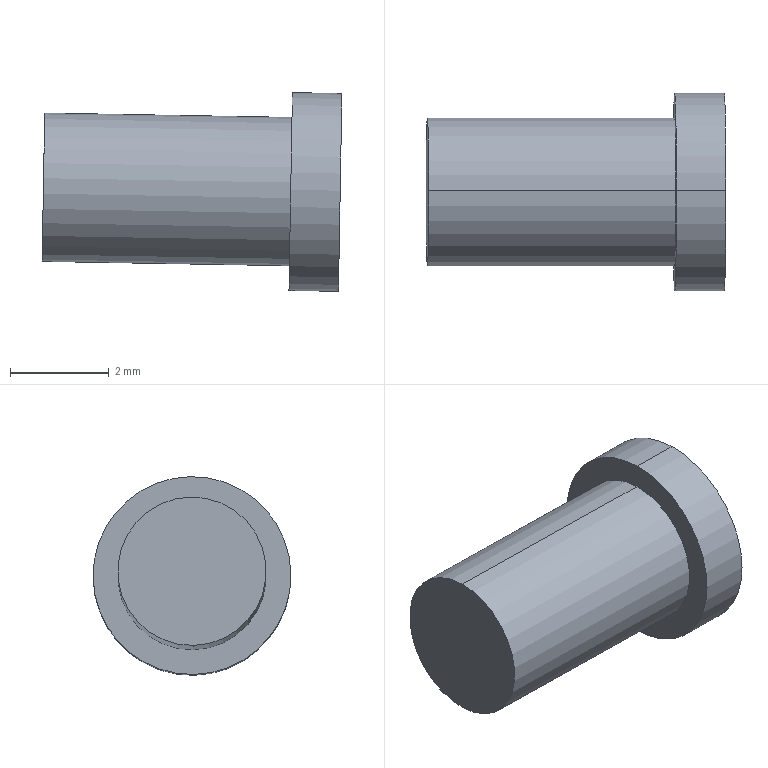Component | SolidWorks | luoding-1 | 1 solid | 7 faces | box 6.06 x 4 x 4.02 mm | volume 48 mm3 | cylinder 4 | plane 3 | commonest cylinder face diameters 4 x2 3 x2
build123d program:
from build123d import *

# Parameters (mm, degrees)
SKETCH1_R           = 1.5
BOSS_EXTRUDE1_DEPTH = 5
SKETCH2_R           = 2
BOSS_EXTRUDE2_DEPTH = 1


with BuildPart() as part:
    # Sketch1 → Boss-Extrude1 (new body)
    with BuildSketch(Plane(origin=(0, 0, 0), x_dir=(1, 0, 0), z_dir=(0, 1, 0))):
        with Locations(Location((0, 0, 0), (0, 0, 270))):
            Circle(SKETCH1_R)
    extrude(amount=BOSS_EXTRUDE1_DEPTH)

    # Sketch2 → Boss-Extrude2 (add)
    with BuildSketch(Plane(origin=(0, 5, 0), x_dir=(1, 0, 0), z_dir=(0, 1, 0))):
        with Locations(Location((0, 0, 0), (0, 0, 270))):
            Circle(SKETCH2_R)
    extrude(amount=BOSS_EXTRUDE2_DEPTH)


solid = part.part

# Placed as in the assembly
solid = solid.moved(Location((23.585, 174.099, 11.545), (92.396, -0.0418, -90.999)))
STEP:
#1=COLOUR_RGB('',0.7922,0.8196,0.9333);
#2=FILL_AREA_STYLE_COLOUR('',#1);
#3=FILL_AREA_STYLE('',(#2));
#4=SURFACE_STYLE_FILL_AREA(#3);
#5=SURFACE_SIDE_STYLE('',(#4));
#6=SURFACE_STYLE_USAGE(.BOTH.,#5);
#7=PRESENTATION_STYLE_ASSIGNMENT((#6));
#8=CARTESIAN_POINT('',(1.166,6.856,0.5291));
#9=VERTEX_POINT('',#8);
#10=CARTESIAN_POINT('',(1.163,6.853,0.3717));
#11=VERTEX_POINT('',#10);
#12=CARTESIAN_POINT('',(1.165,6.854,0.4504));
#13=DIRECTION('',(0.9998,0.,-0.01745));
#14=DIRECTION('',(0.01745,0.01745,0.9997));
#15=AXIS2_PLACEMENT_3D('',#12,#13,#14);
#16=CIRCLE('',#15,0.07874);
#17=EDGE_CURVE('',#9,#11,#16,.T.);
#18=ORIENTED_EDGE('',*,*,#17,.F.);
#19=CARTESIAN_POINT('',(1.127,6.856,0.5298));
#20=VERTEX_POINT('',#19);
#21=CARTESIAN_POINT('',(1.166,6.856,0.5291));
#22=DIRECTION('',(-0.9998,-0.,0.01745));
#23=VECTOR('',#22,39.37);
#24=LINE('',#21,#23);
#25=EDGE_CURVE('',#9,#20,#24,.T.);
#26=ORIENTED_EDGE('',*,*,#25,.T.);
#27=CARTESIAN_POINT('',(1.124,6.853,0.3724));
#28=VERTEX_POINT('',#27);
#29=CARTESIAN_POINT('',(1.125,6.854,0.4511));
#30=DIRECTION('',(0.9998,0.,-0.01745));
#31=DIRECTION('',(0.01745,0.01745,0.9997));
#32=AXIS2_PLACEMENT_3D('',#29,#30,#31);
#33=CIRCLE('',#32,0.07874);
#34=EDGE_CURVE('',#20,#28,#33,.T.);
#35=ORIENTED_EDGE('',*,*,#34,.T.);
#36=CARTESIAN_POINT('',(1.163,6.853,0.3717));
#37=DIRECTION('',(-0.9998,-0.,0.01745));
#38=VECTOR('',#37,39.37);
#39=LINE('',#36,#38);
#40=EDGE_CURVE('',#11,#28,#39,.T.);
#41=ORIENTED_EDGE('',*,*,#40,.F.);
#42=EDGE_LOOP('',(#18,#26,#35,#41));
#43=FACE_OUTER_BOUND('',#42,.T.);
#44=CARTESIAN_POINT('',(1.165,6.854,0.4504));
#45=DIRECTION('',(-0.9998,-0.,0.01745));
#46=DIRECTION('',(-0.01745,-0.01745,-0.9997));
#47=AXIS2_PLACEMENT_3D('',#44,#45,#46);
#48=CYLINDRICAL_SURFACE('',#47,0.07874);
#49=ADVANCED_FACE('',(#43),#48,.T.);
#50=CARTESIAN_POINT('',(1.126,6.855,0.5101));
#51=VERTEX_POINT('',#50);
#52=CARTESIAN_POINT('',(1.124,6.853,0.3921));
#53=VERTEX_POINT('',#52);
#54=CARTESIAN_POINT('',(1.125,6.854,0.4511));
#55=DIRECTION('',(0.9998,0.,-0.01745));
#56=DIRECTION('',(0.01745,0.01745,0.9997));
#57=AXIS2_PLACEMENT_3D('',#54,#55,#56);
#58=CIRCLE('',#57,0.05906);
#59=EDGE_CURVE('',#51,#53,#58,.T.);
#60=ORIENTED_EDGE('',*,*,#59,.F.);
#61=CARTESIAN_POINT('',(0.9296,6.855,0.5136));
#62=VERTEX_POINT('',#61);
#63=CARTESIAN_POINT('',(1.126,6.855,0.5101));
#64=DIRECTION('',(-0.9998,-0.,0.01745));
#65=VECTOR('',#64,39.37);
#66=LINE('',#63,#65);
#67=EDGE_CURVE('',#51,#62,#66,.T.);
#68=ORIENTED_EDGE('',*,*,#67,.T.);
#69=CARTESIAN_POINT('',(0.9275,6.853,0.3955));
#70=VERTEX_POINT('',#69);
#71=CARTESIAN_POINT('',(0.9285,6.854,0.4545));
#72=DIRECTION('',(0.9998,0.,-0.01745));
#73=DIRECTION('',(0.01745,0.01745,0.9997));
#74=AXIS2_PLACEMENT_3D('',#71,#72,#73);
#75=CIRCLE('',#74,0.05906);
#76=EDGE_CURVE('',#62,#70,#75,.T.);
#77=ORIENTED_EDGE('',*,*,#76,.T.);
#78=CARTESIAN_POINT('',(1.124,6.853,0.3921));
#79=DIRECTION('',(-0.9998,-0.,0.01745));
#80=VECTOR('',#79,39.37);
#81=LINE('',#78,#80);
#82=EDGE_CURVE('',#53,#70,#81,.T.);
#83=ORIENTED_EDGE('',*,*,#82,.F.);
#84=EDGE_LOOP('',(#60,#68,#77,#83));
#85=FACE_OUTER_BOUND('',#84,.T.);
#86=CARTESIAN_POINT('',(1.125,6.854,0.4511));
#87=DIRECTION('',(-0.9998,-0.,0.01745));
#88=DIRECTION('',(-0.01745,-0.01745,-0.9997));
#89=AXIS2_PLACEMENT_3D('',#86,#87,#88);
#90=CYLINDRICAL_SURFACE('',#89,0.05906);
#91=ADVANCED_FACE('',(#85),#90,.T.);
#92=ORIENTED_EDGE('',*,*,#67,.F.);
#93=CARTESIAN_POINT('',(1.125,6.854,0.4511));
#94=DIRECTION('',(0.9998,0.,-0.01745));
#95=DIRECTION('',(0.01745,0.01745,0.9997));
#96=AXIS2_PLACEMENT_3D('',#93,#94,#95);
#97=CIRCLE('',#96,0.05906);
#98=EDGE_CURVE('',#53,#51,#97,.T.);
#99=ORIENTED_EDGE('',*,*,#98,.F.);
#100=ORIENTED_EDGE('',*,*,#82,.T.);
#101=CARTESIAN_POINT('',(0.9285,6.854,0.4545));
#102=DIRECTION('',(0.9998,0.,-0.01745));
#103=DIRECTION('',(0.01745,0.01745,0.9997));
#104=AXIS2_PLACEMENT_3D('',#101,#102,#103);
#105=CIRCLE('',#104,0.05906);
#106=EDGE_CURVE('',#70,#62,#105,.T.);
#107=ORIENTED_EDGE('',*,*,#106,.T.);
#108=EDGE_LOOP('',(#92,#99,#100,#107));
#109=FACE_OUTER_BOUND('',#108,.T.);
#110=CARTESIAN_POINT('',(1.125,6.854,0.4511));
#111=DIRECTION('',(-0.9998,-0.,0.01745));
#112=DIRECTION('',(-0.01745,-0.01745,-0.9997));
#113=AXIS2_PLACEMENT_3D('',#110,#111,#112);
#114=CYLINDRICAL_SURFACE('',#113,0.05906);
#115=ADVANCED_FACE('',(#109),#114,.T.);
#116=ORIENTED_EDGE('',*,*,#106,.F.);
#117=ORIENTED_EDGE('',*,*,#76,.F.);
#118=EDGE_LOOP('',(#116,#117));
#119=FACE_OUTER_BOUND('',#118,.T.);
#120=CARTESIAN_POINT('',(0.9285,6.854,0.4545));
#121=DIRECTION('',(0.9998,0.,-0.01745));
#122=DIRECTION('',(0.01745,0.01745,0.9997));
#123=AXIS2_PLACEMENT_3D('',#120,#121,#122);
#124=PLANE('',#123);
#125=ADVANCED_FACE('',(#119),#124,.F.);
#126=ORIENTED_EDGE('',*,*,#25,.F.);
#127=CARTESIAN_POINT('',(1.165,6.854,0.4504));
#128=DIRECTION('',(0.9998,0.,-0.01745));
#129=DIRECTION('',(0.01745,0.01745,0.9997));
#130=AXIS2_PLACEMENT_3D('',#127,#128,#129);
#131=CIRCLE('',#130,0.07874);
#132=EDGE_CURVE('',#11,#9,#131,.T.);
#133=ORIENTED_EDGE('',*,*,#132,.F.);
#134=ORIENTED_EDGE('',*,*,#40,.T.);
#135=CARTESIAN_POINT('',(1.125,6.854,0.4511));
#136=DIRECTION('',(0.9998,0.,-0.01745));
#137=DIRECTION('',(0.01745,0.01745,0.9997));
#138=AXIS2_PLACEMENT_3D('',#135,#136,#137);
#139=CIRCLE('',#138,0.07874);
#140=EDGE_CURVE('',#28,#20,#139,.T.);
#141=ORIENTED_EDGE('',*,*,#140,.T.);
#142=EDGE_LOOP('',(#126,#133,#134,#141));
#143=FACE_OUTER_BOUND('',#142,.T.);
#144=CARTESIAN_POINT('',(1.165,6.854,0.4504));
#145=DIRECTION('',(-0.9998,-0.,0.01745));
#146=DIRECTION('',(-0.01745,-0.01745,-0.9997));
#147=AXIS2_PLACEMENT_3D('',#144,#145,#146);
#148=CYLINDRICAL_SURFACE('',#147,0.07874);
#149=ADVANCED_FACE('',(#143),#148,.T.);
#150=ORIENTED_EDGE('',*,*,#132,.T.);
#151=ORIENTED_EDGE('',*,*,#17,.T.);
#152=EDGE_LOOP('',(#150,#151));
#153=FACE_OUTER_BOUND('',#152,.T.);
#154=CARTESIAN_POINT('',(1.165,6.854,0.4504));
#155=DIRECTION('',(0.9998,0.,-0.01745));
#156=DIRECTION('',(0.01745,0.01745,0.9997));
#157=AXIS2_PLACEMENT_3D('',#154,#155,#156);
#158=PLANE('',#157);
#159=ADVANCED_FACE('',(#153),#158,.T.);
#160=ORIENTED_EDGE('',*,*,#98,.T.);
#161=ORIENTED_EDGE('',*,*,#59,.T.);
#162=EDGE_LOOP('',(#160,#161));
#163=FACE_BOUND('',#162,.T.);
#164=ORIENTED_EDGE('',*,*,#140,.F.);
#165=ORIENTED_EDGE('',*,*,#34,.F.);
#166=EDGE_LOOP('',(#164,#165));
#167=FACE_OUTER_BOUND('',#166,.T.);
#168=CARTESIAN_POINT('',(1.125,6.854,0.4511));
#169=DIRECTION('',(0.9998,0.,-0.01745));
#170=DIRECTION('',(0.01745,0.01745,0.9997));
#171=AXIS2_PLACEMENT_3D('',#168,#169,#170);
#172=PLANE('',#171);
#173=ADVANCED_FACE('',(#163,#167),#172,.F.);
#174=CLOSED_SHELL('',(#49,#91,#115,#125,#149,#159,#173));
#175=MANIFOLD_SOLID_BREP('',#174);
#176=STYLED_ITEM('',(#7),#175);
#177=PRESENTATION_LAYER_ASSIGNMENT('','',(#176));
#178=CARTESIAN_POINT('',(0.,0.,0.));
#179=DIRECTION('',(0.,0.,1.));
#180=DIRECTION('',(1.,0.,0.));
#181=AXIS2_PLACEMENT_3D('',#178,#179,#180);
#182=(LENGTH_UNIT()NAMED_UNIT(*)SI_UNIT($,.METRE.));
#183=LENGTH_MEASURE_WITH_UNIT(LENGTH_MEASURE(0.0254),#182);
#184=DIMENSIONAL_EXPONENTS(1.,0.,0.,0.,0.,0.,0.);
#185=(CONVERSION_BASED_UNIT('',#183)LENGTH_UNIT()NAMED_UNIT(#184));
#186=UNCERTAINTY_MEASURE_WITH_UNIT(LENGTH_MEASURE(0.00001),#185,'','');
#187=(NAMED_UNIT(*)PLANE_ANGLE_UNIT()SI_UNIT($,.RADIAN.));
#188=(NAMED_UNIT(*)SI_UNIT($,.STERADIAN.)SOLID_ANGLE_UNIT());
#189=(GEOMETRIC_REPRESENTATION_CONTEXT(3)GLOBAL_UNCERTAINTY_ASSIGNED_CONTEXT((#186))GLOBAL_UNIT_ASSIGNED_CONTEXT((#185,#187,#188))REPRESENTATION_CONTEXT('',''));
#190=ADVANCED_BREP_SHAPE_REPRESENTATION('',(#175,#181),#189);
#191=(LENGTH_UNIT()NAMED_UNIT(*)SI_UNIT($,.METRE.));
#192=LENGTH_MEASURE_WITH_UNIT(LENGTH_MEASURE(0.0254),#191);
#193=DIMENSIONAL_EXPONENTS(1.,0.,0.,0.,0.,0.,0.);
#194=(CONVERSION_BASED_UNIT('',#192)LENGTH_UNIT()NAMED_UNIT(#193));
#195=UNCERTAINTY_MEASURE_WITH_UNIT(LENGTH_MEASURE(0.00001),#194,'','');
#196=(NAMED_UNIT(*)PLANE_ANGLE_UNIT()SI_UNIT($,.RADIAN.));
#197=(NAMED_UNIT(*)SI_UNIT($,.STERADIAN.)SOLID_ANGLE_UNIT());
#198=(GEOMETRIC_REPRESENTATION_CONTEXT(3)GLOBAL_UNCERTAINTY_ASSIGNED_CONTEXT((#195))GLOBAL_UNIT_ASSIGNED_CONTEXT((#194,#196,#197))REPRESENTATION_CONTEXT('',''));
#199=MECHANICAL_DESIGN_GEOMETRIC_PRESENTATION_REPRESENTATION('',(#176),#198);